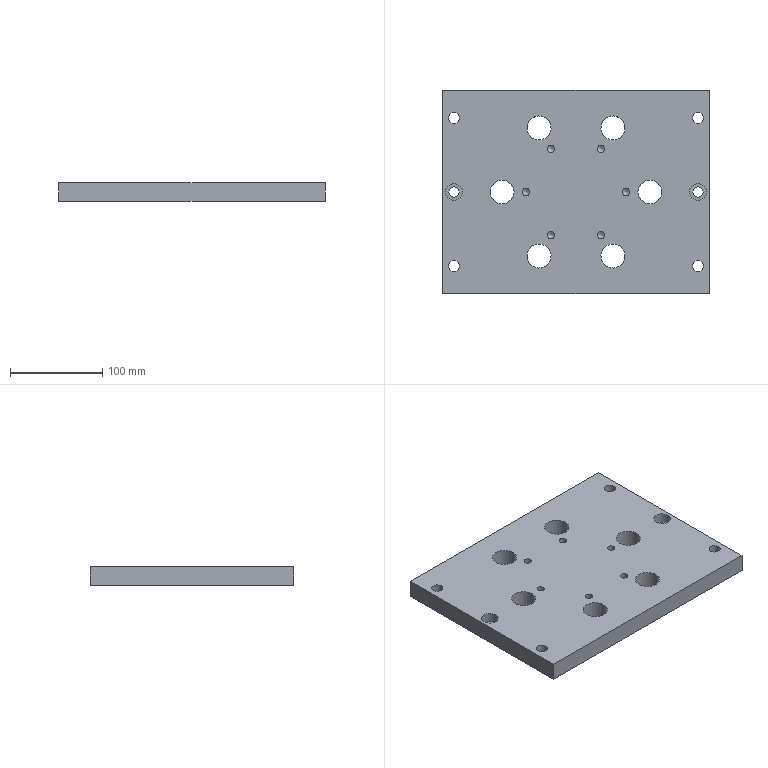Component | NX | DRILL_TEMPLATE | 1 solid | 34 faces | volume 1182128 mm3 | cylinder 20 | plane 8 | cone 6 | commonest cylinder face diameters 26 x6 8 x6 12 x4 11 x2 18 x2